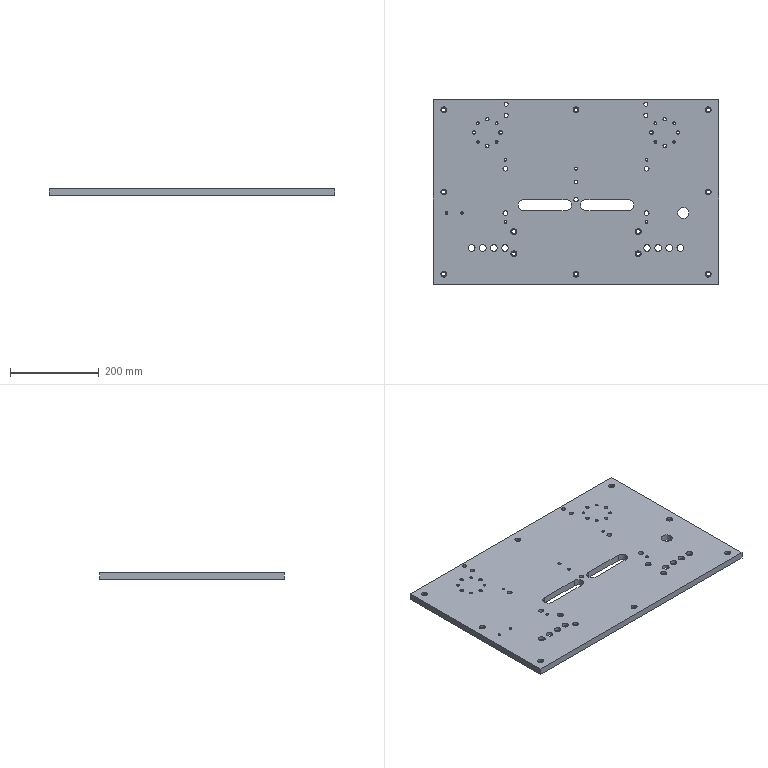Component | SolidWorks | FrameAssembly-1_LongitudinalSealPanel-1 | 1 solid | 216 faces | volume 3824896 mm3 | cylinder 144 | cone 44 | plane 28 | commonest cylinder face diameters 9 x32 5 x28 13.5 x24 6.8 x16 15 x16 11 x8 25 x8 26 x6